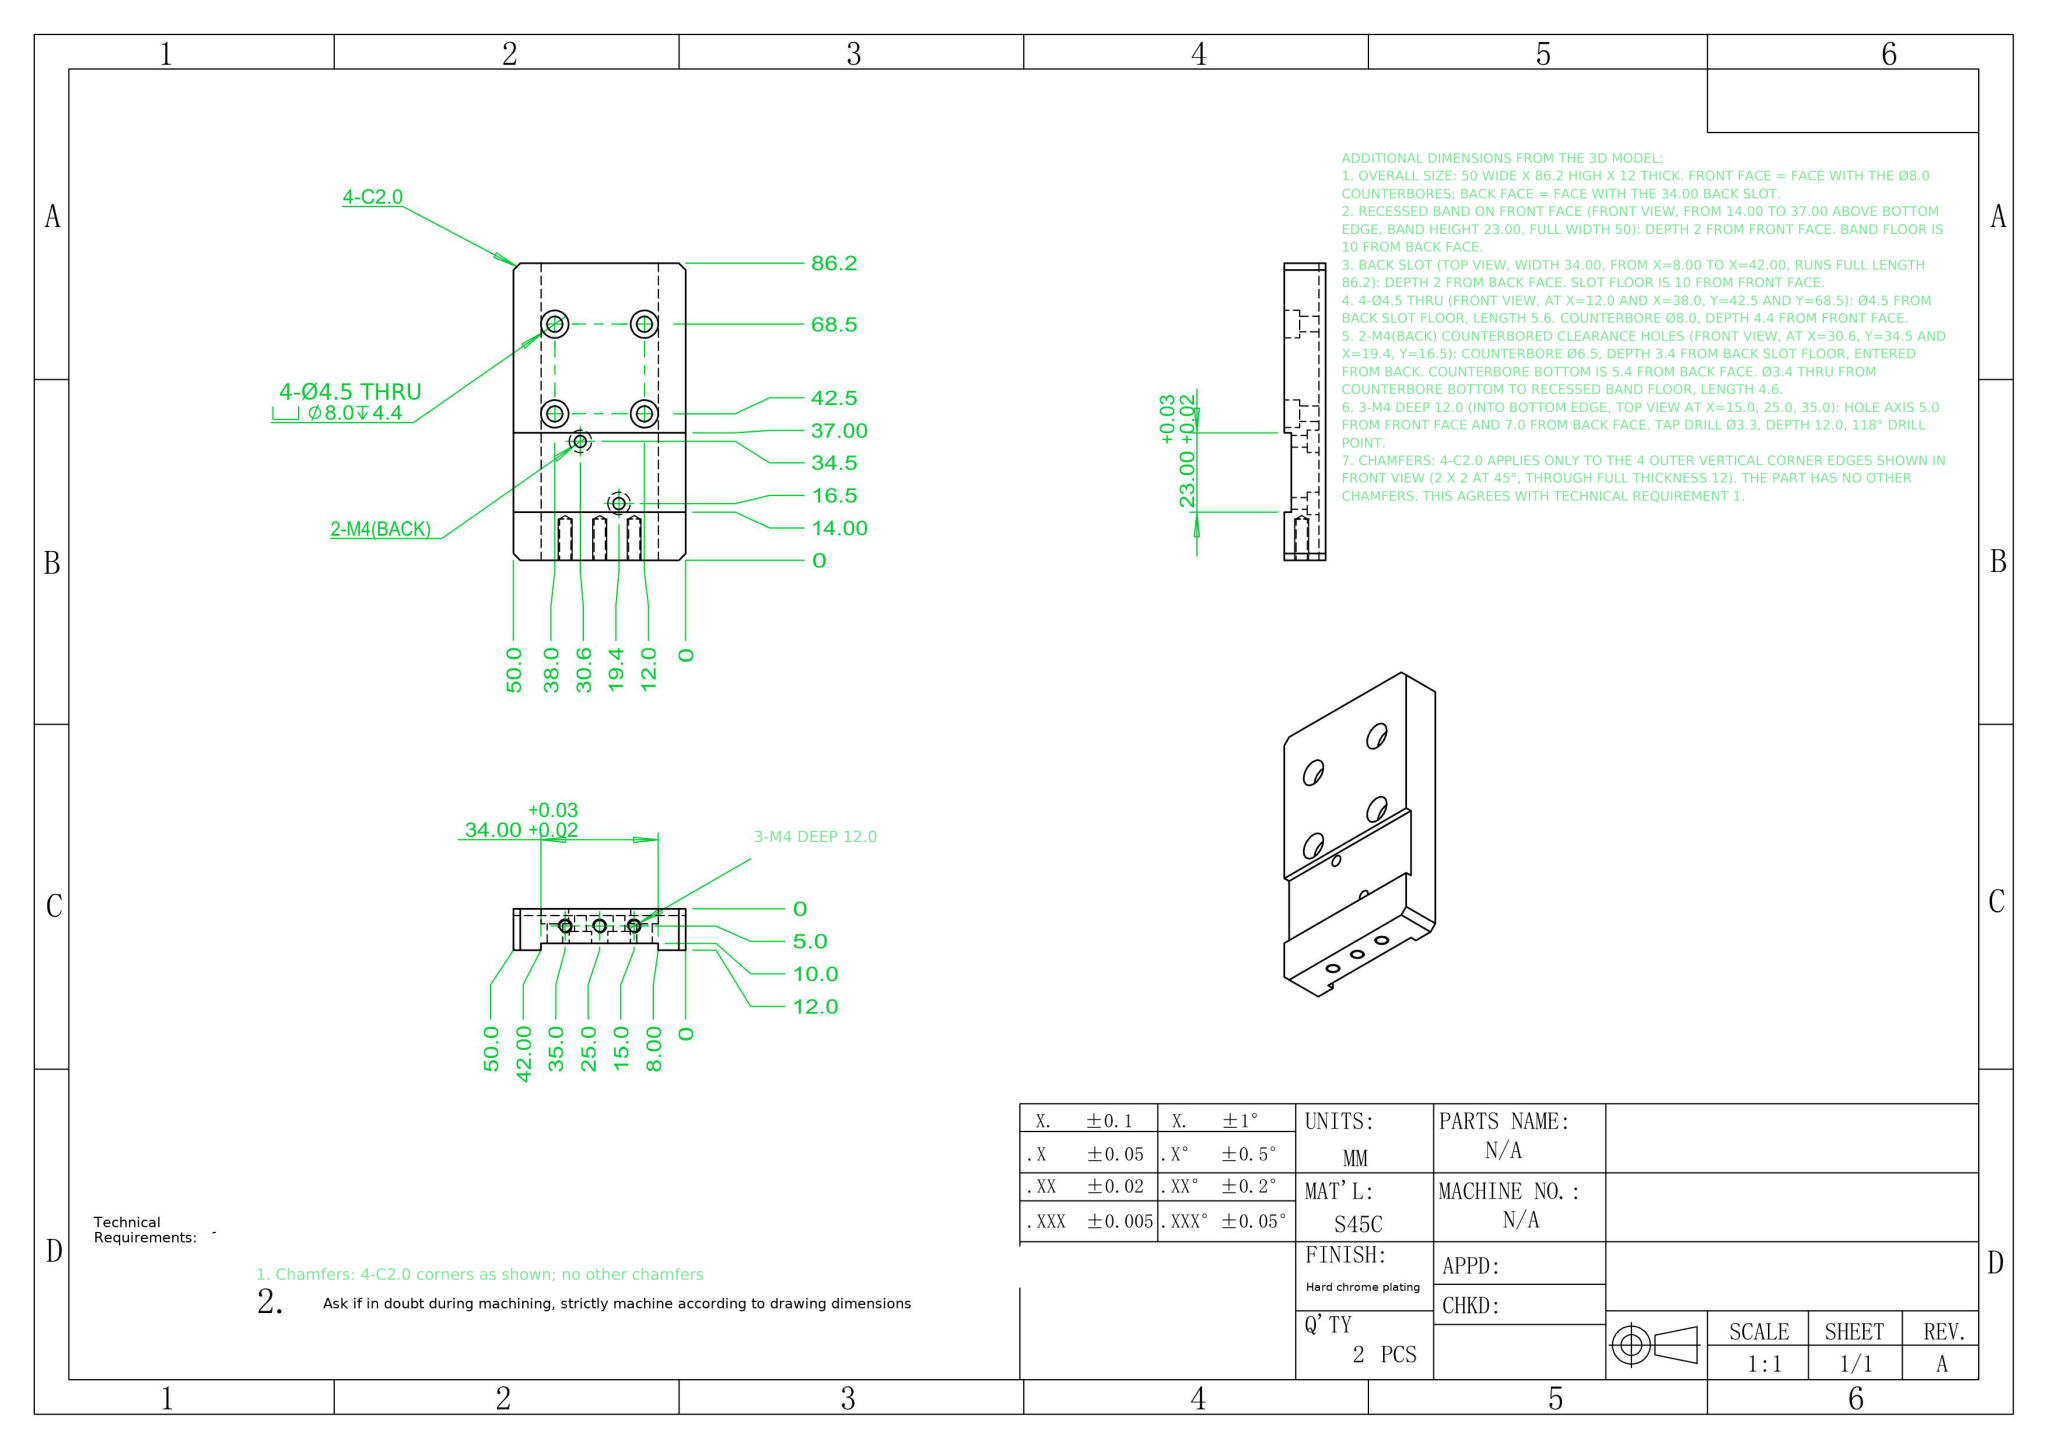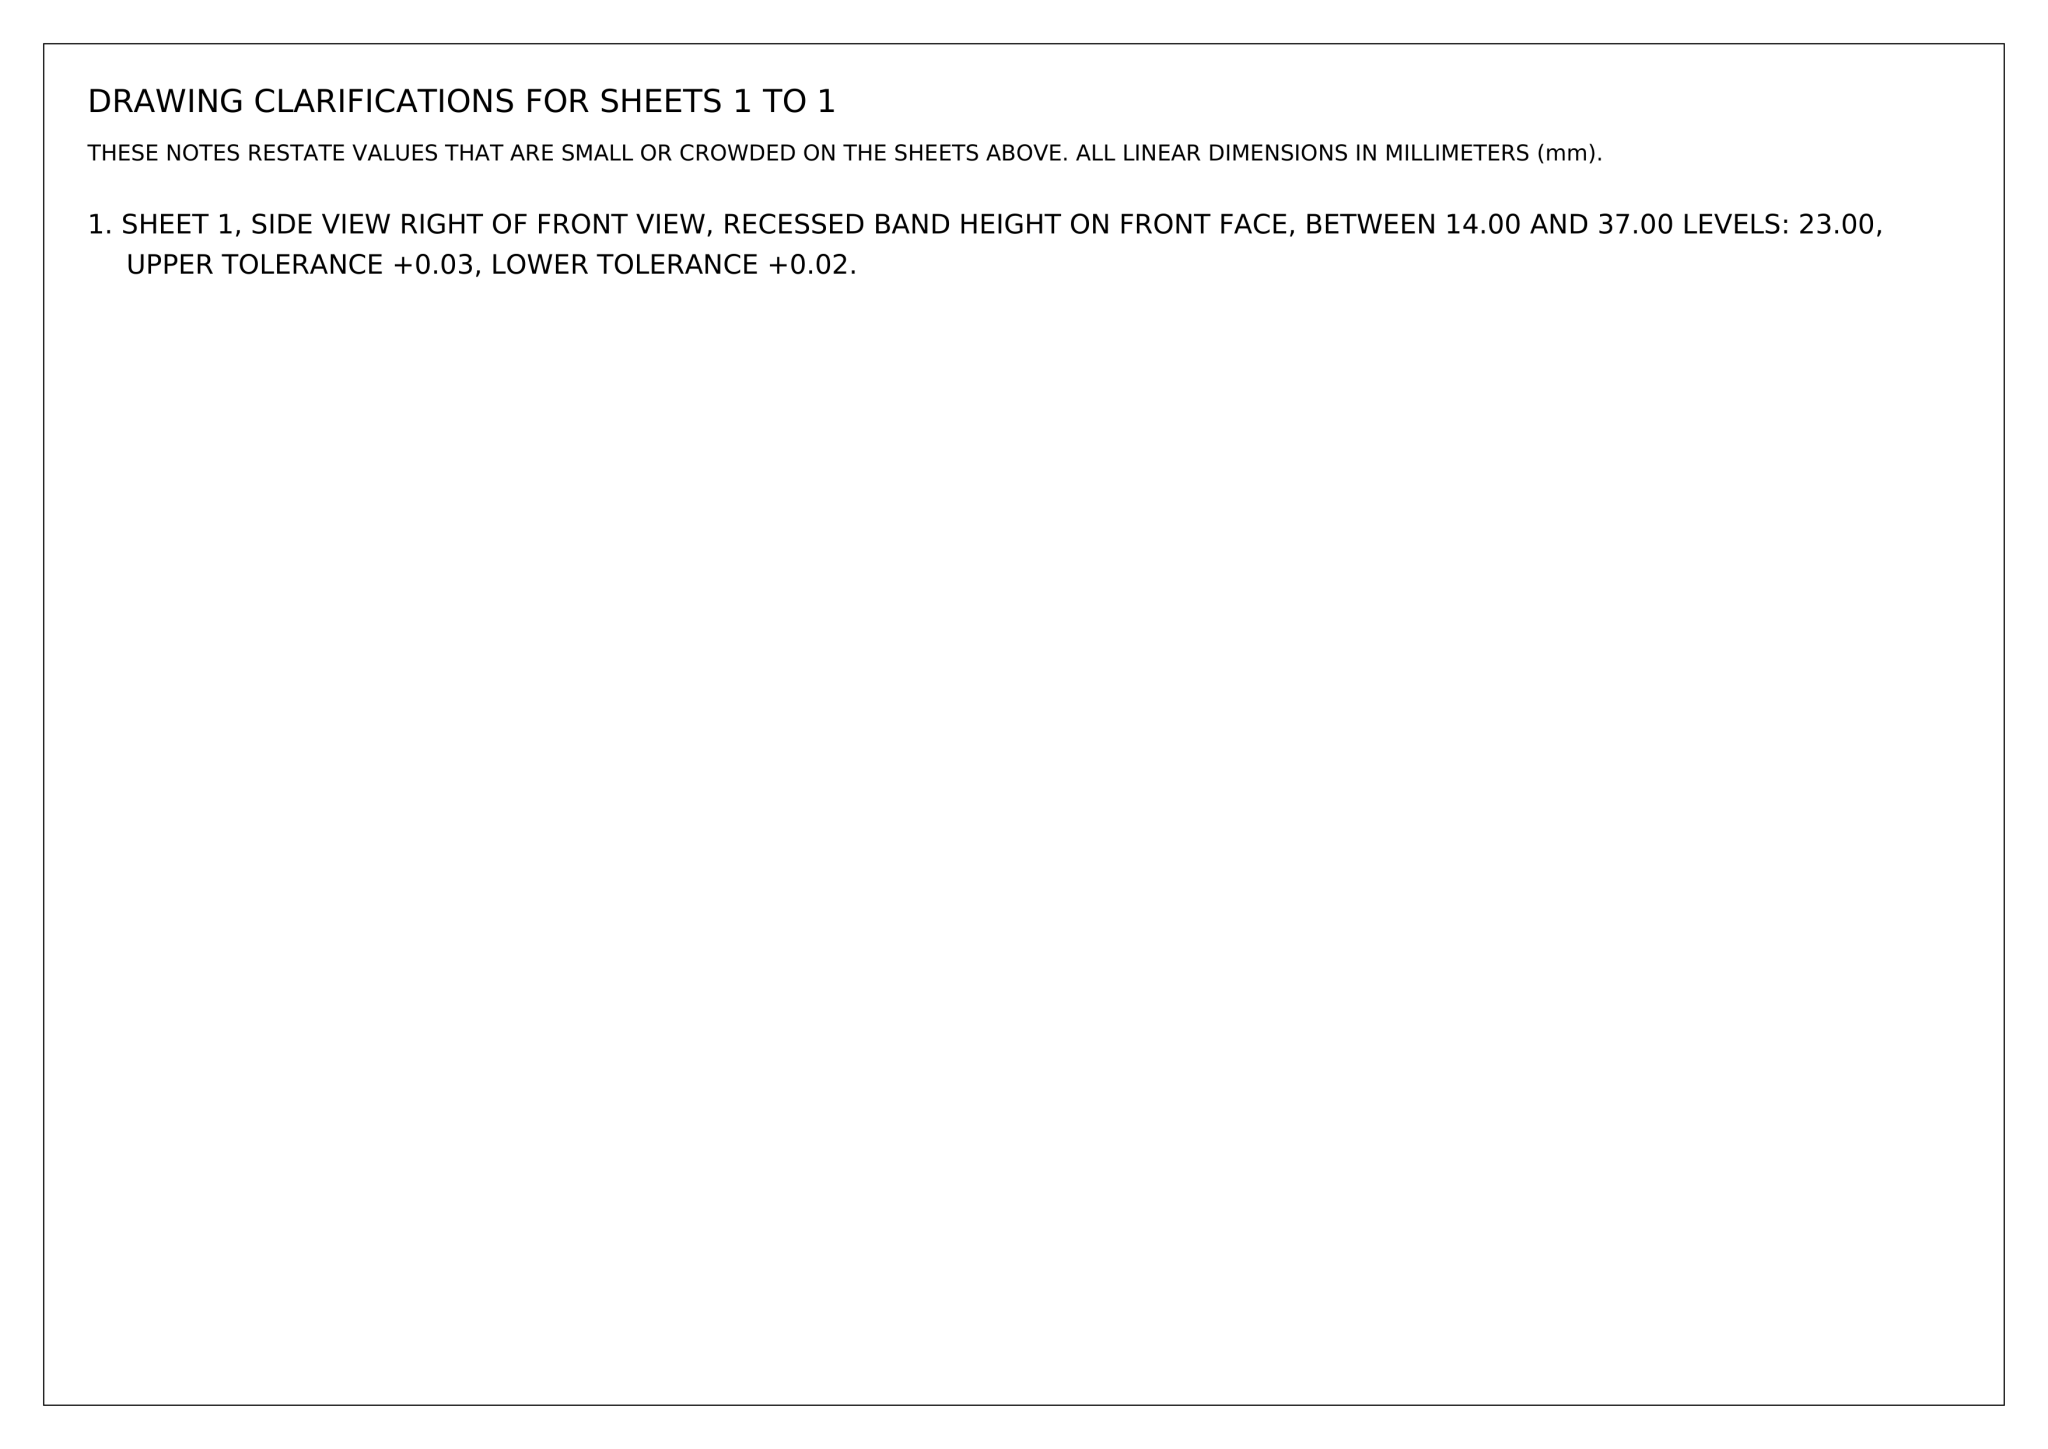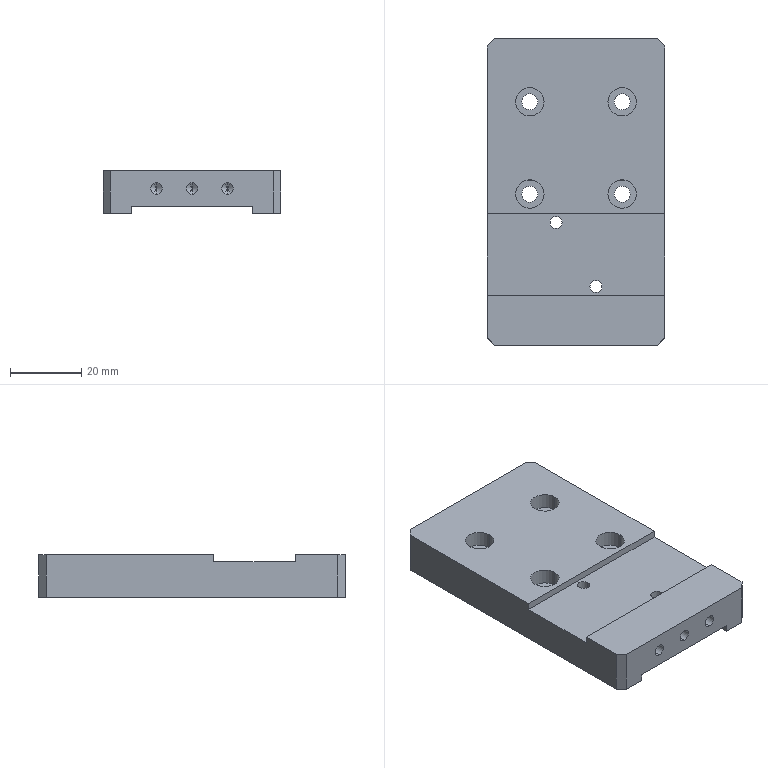Part | NX | mm | 1 solid | 60 faces | box 50 x 86.2 x 12 mm | volume 41596 mm3 | cylinder 30 | plane 24 | cone 6 | commonest cylinder face diameters 8 x8 4.5 x8 3.3 x6 6.5 x4 3.4 x4